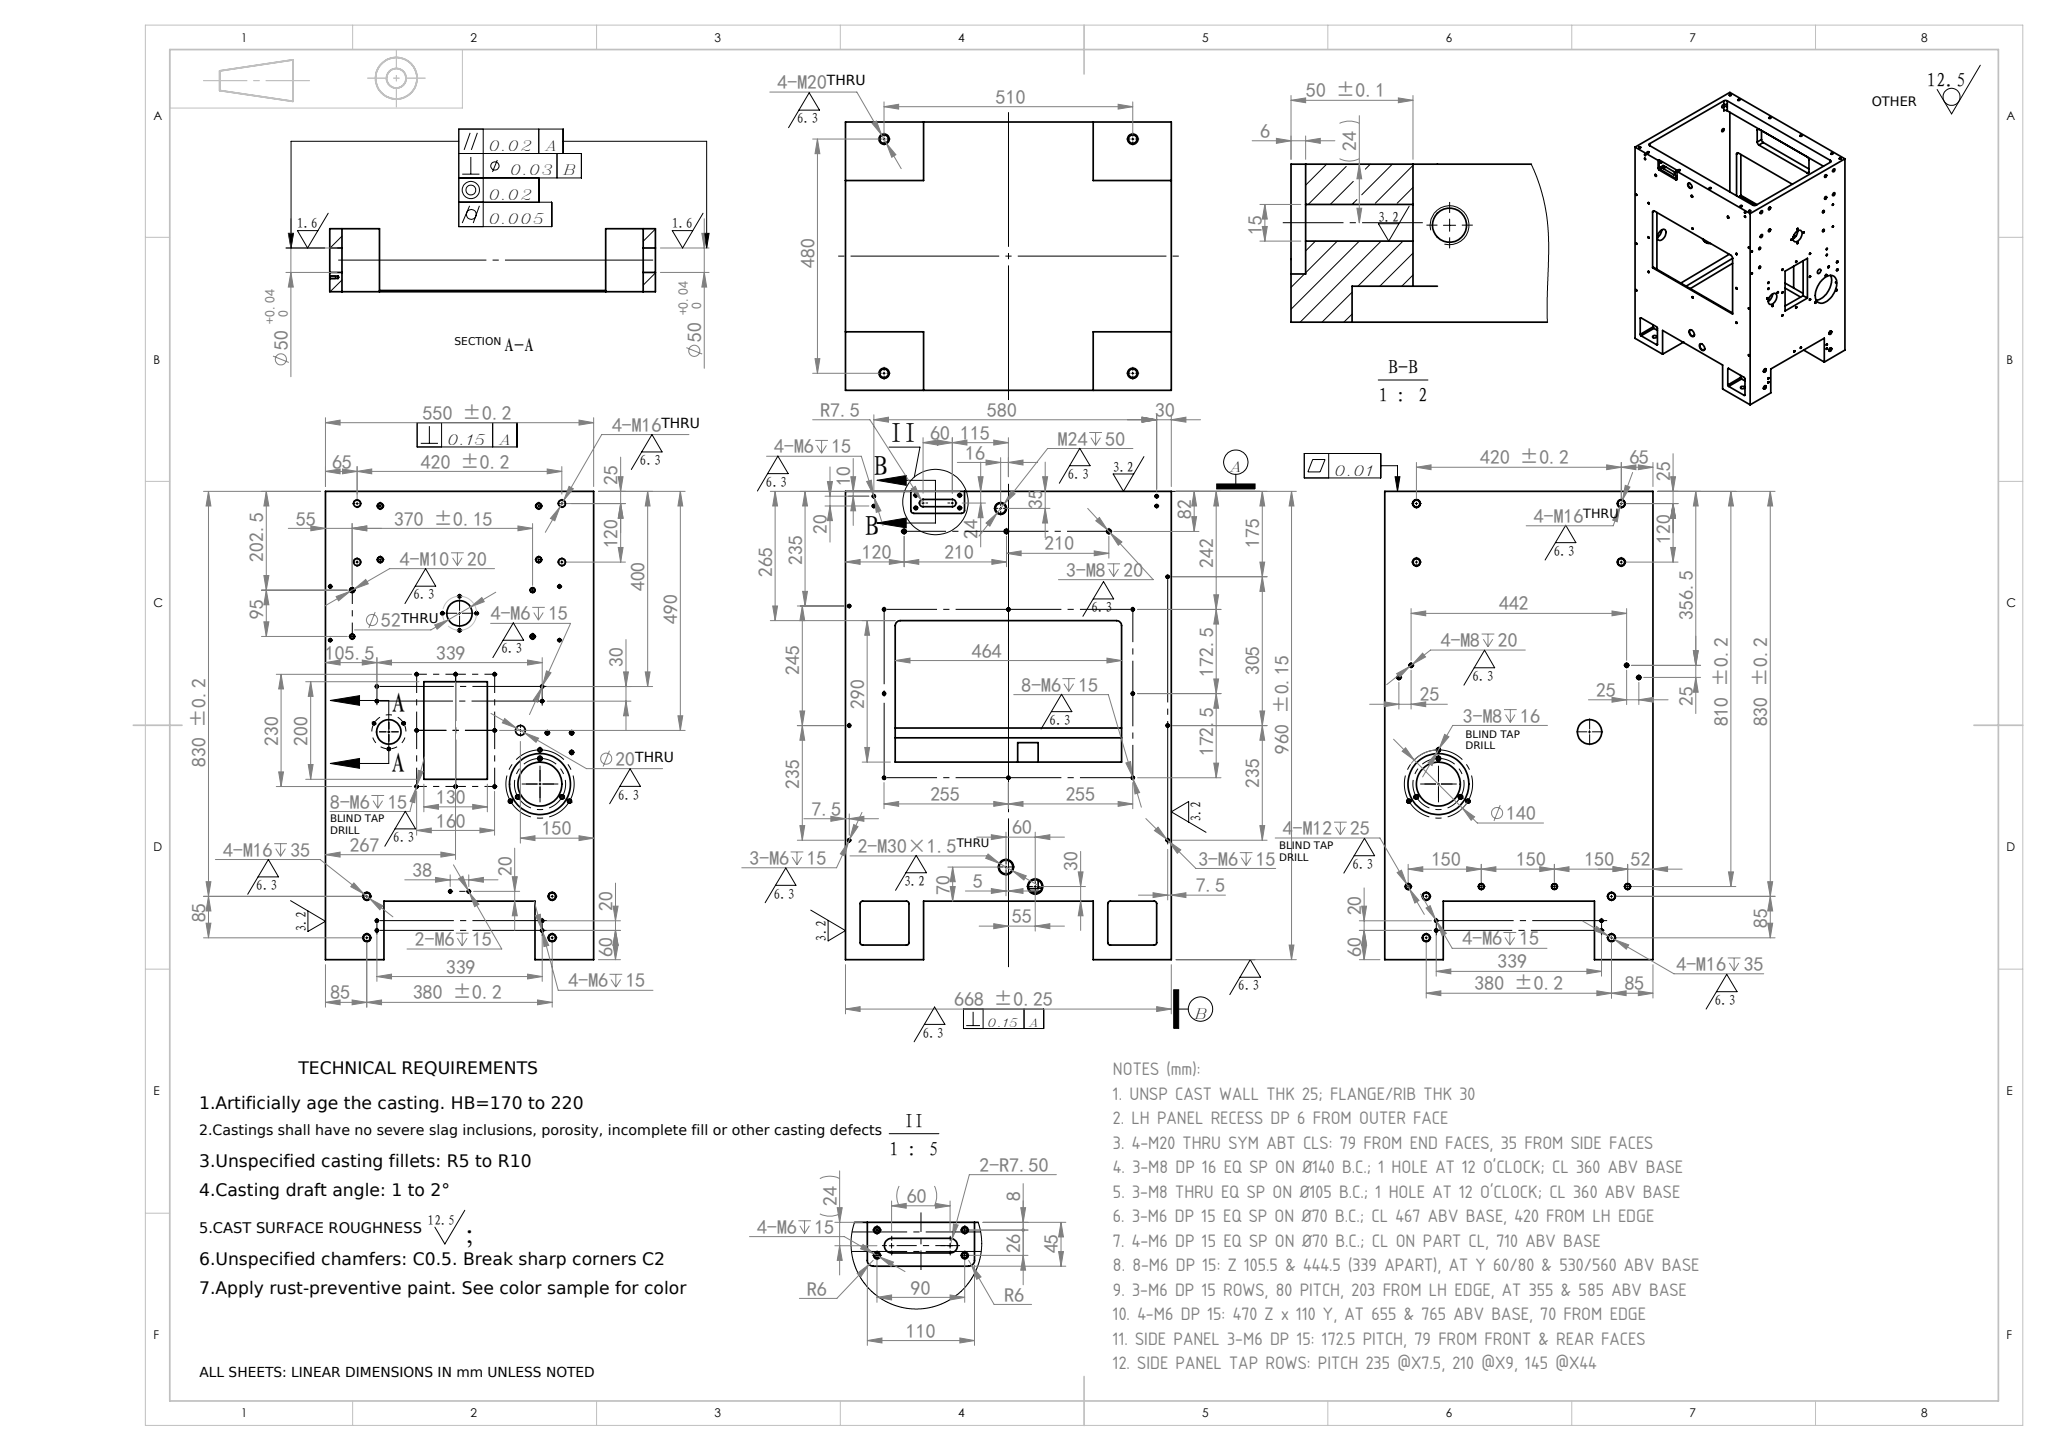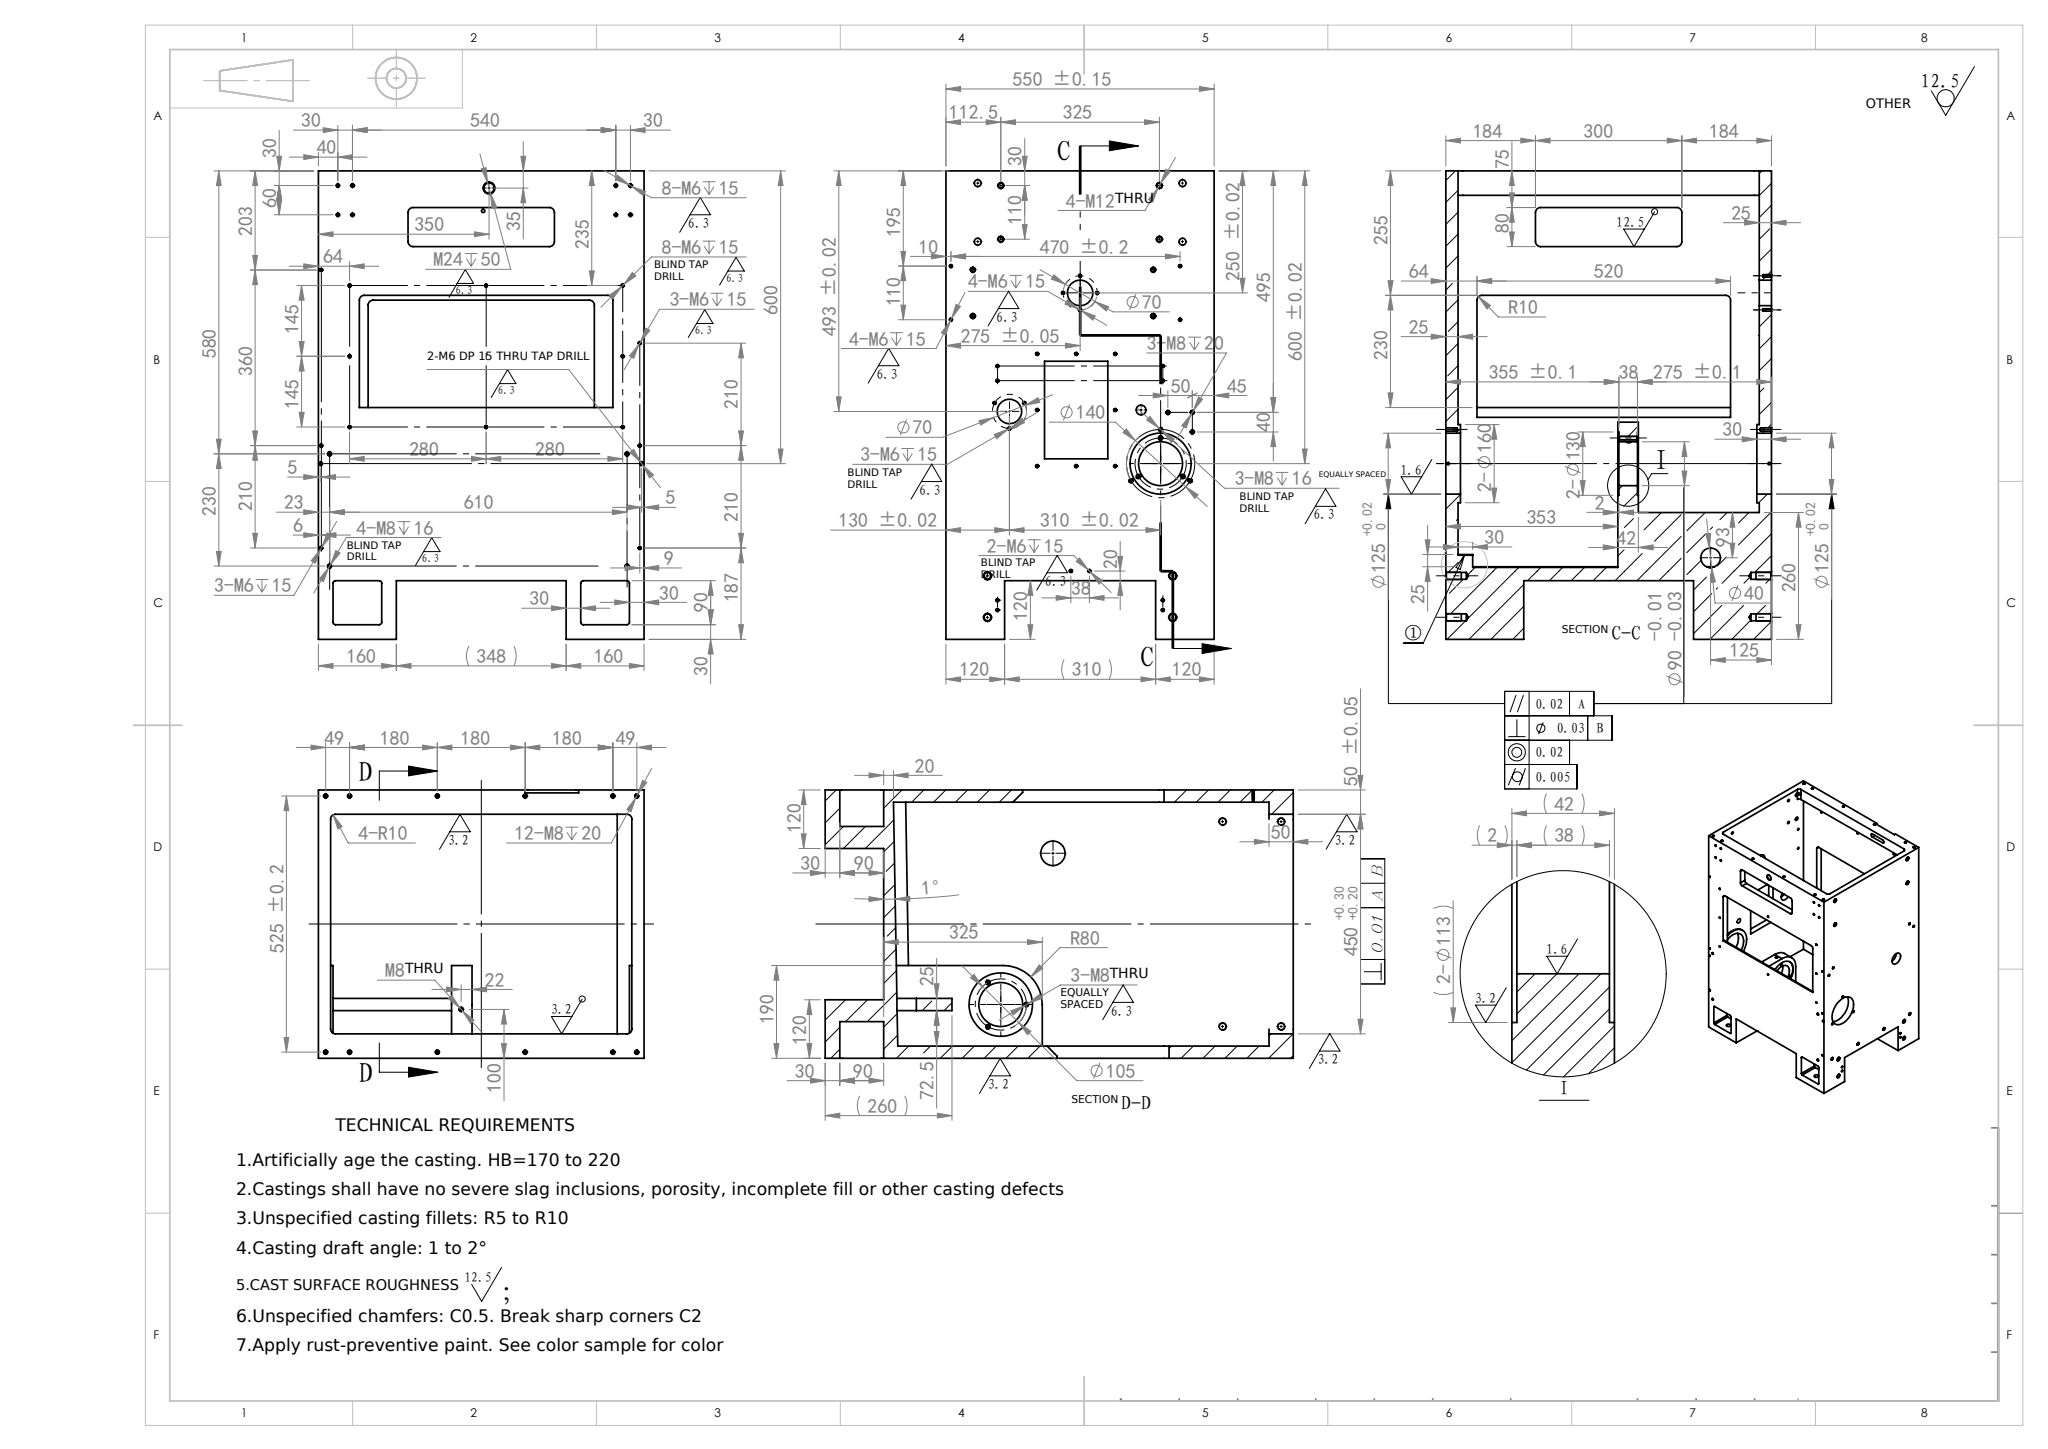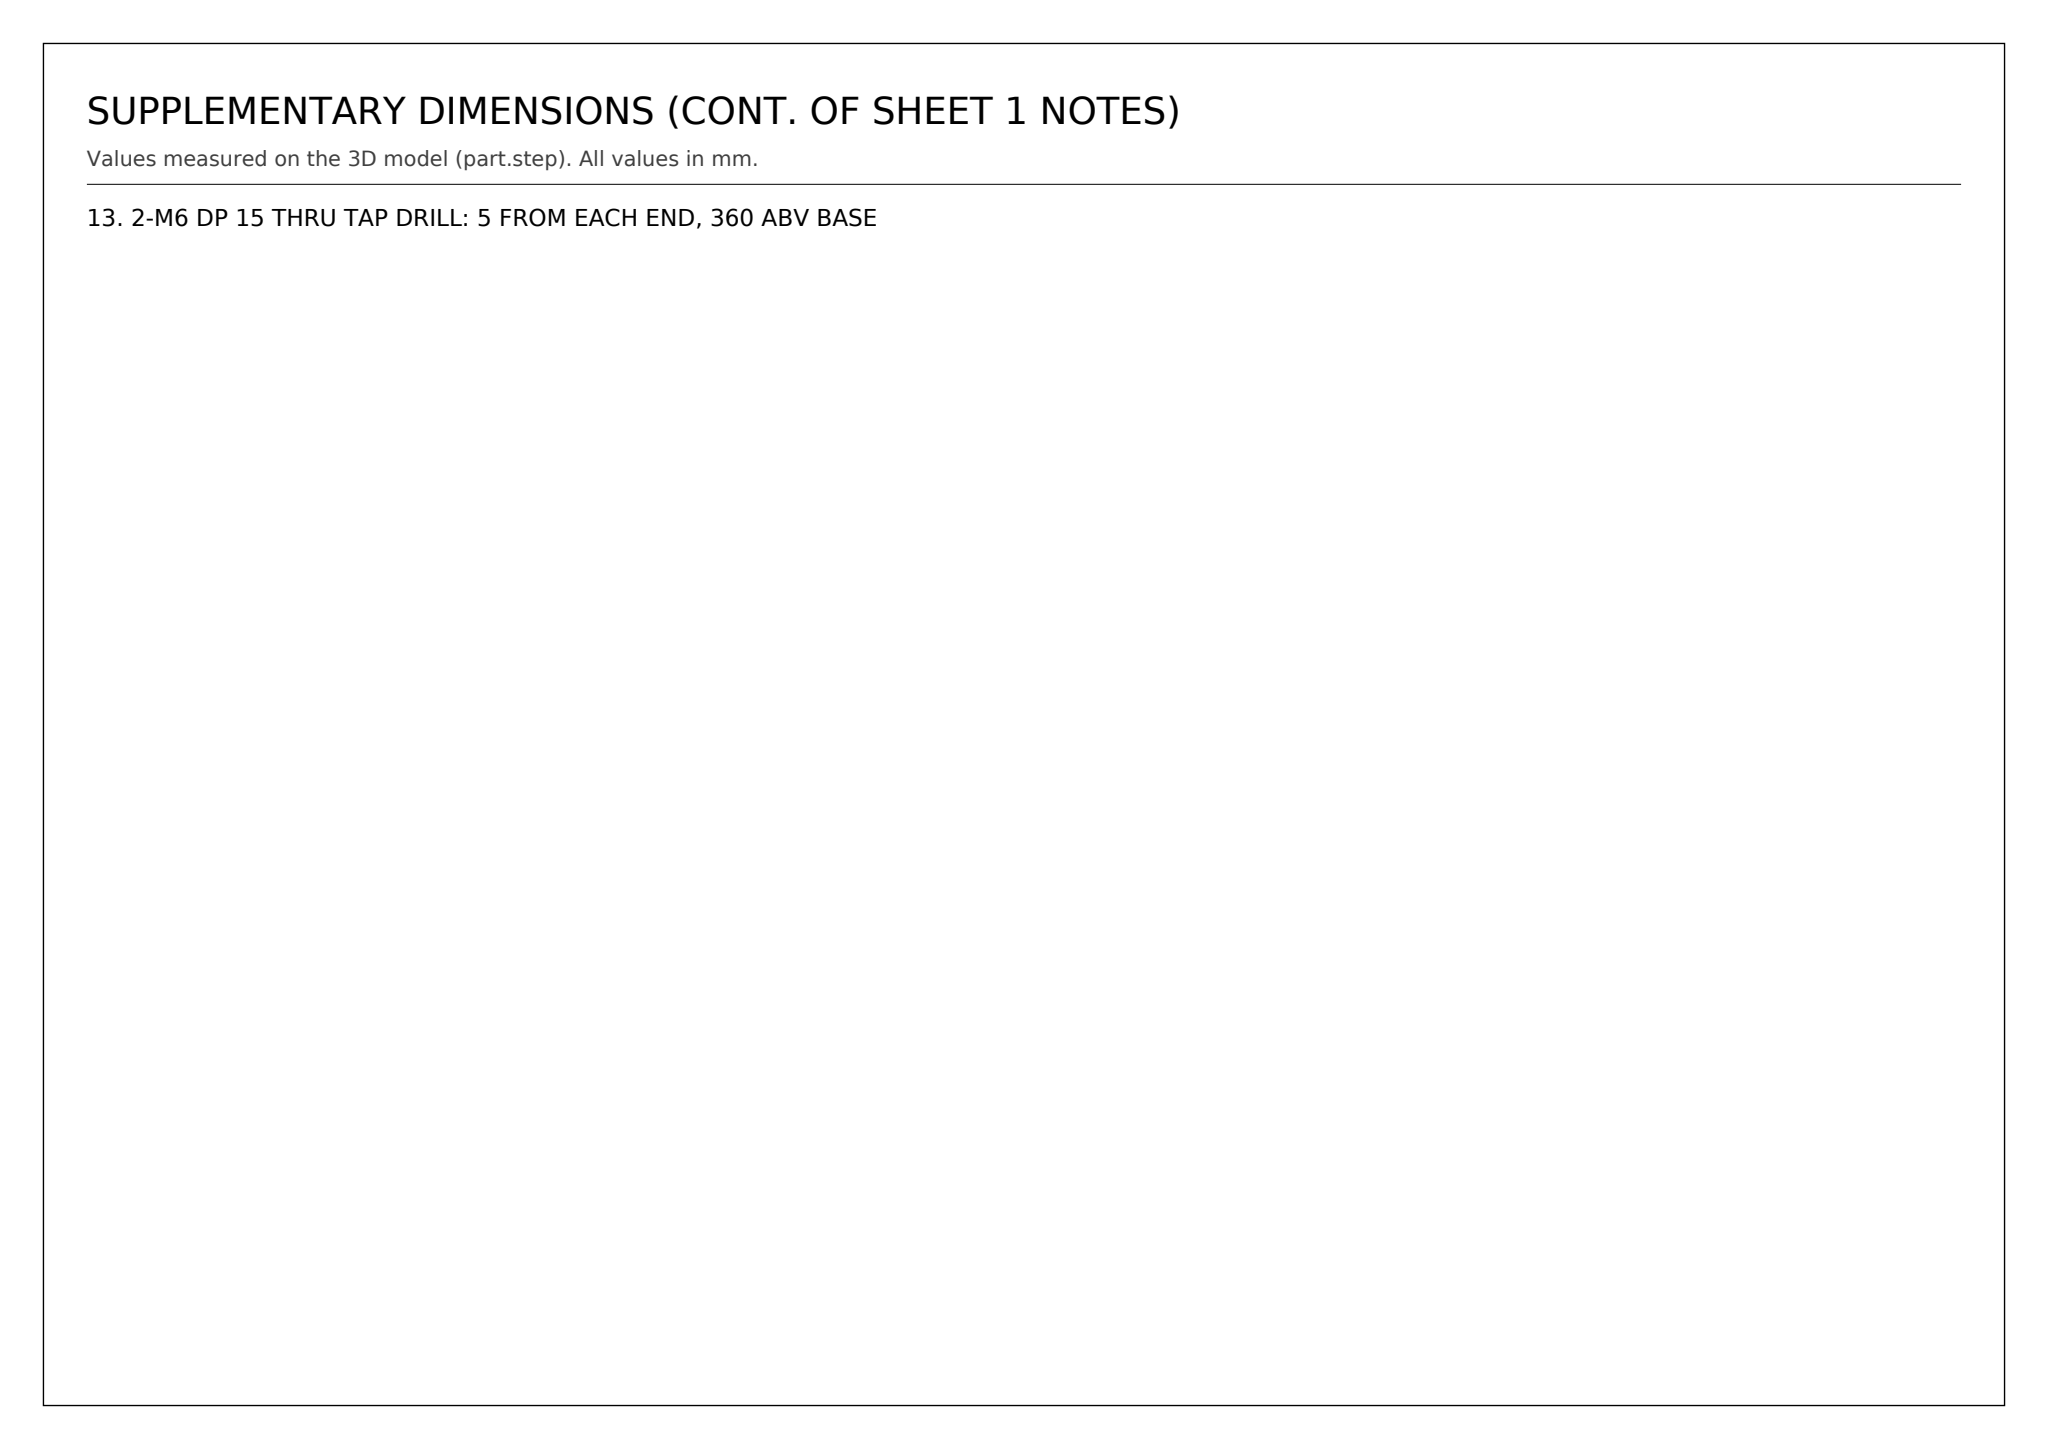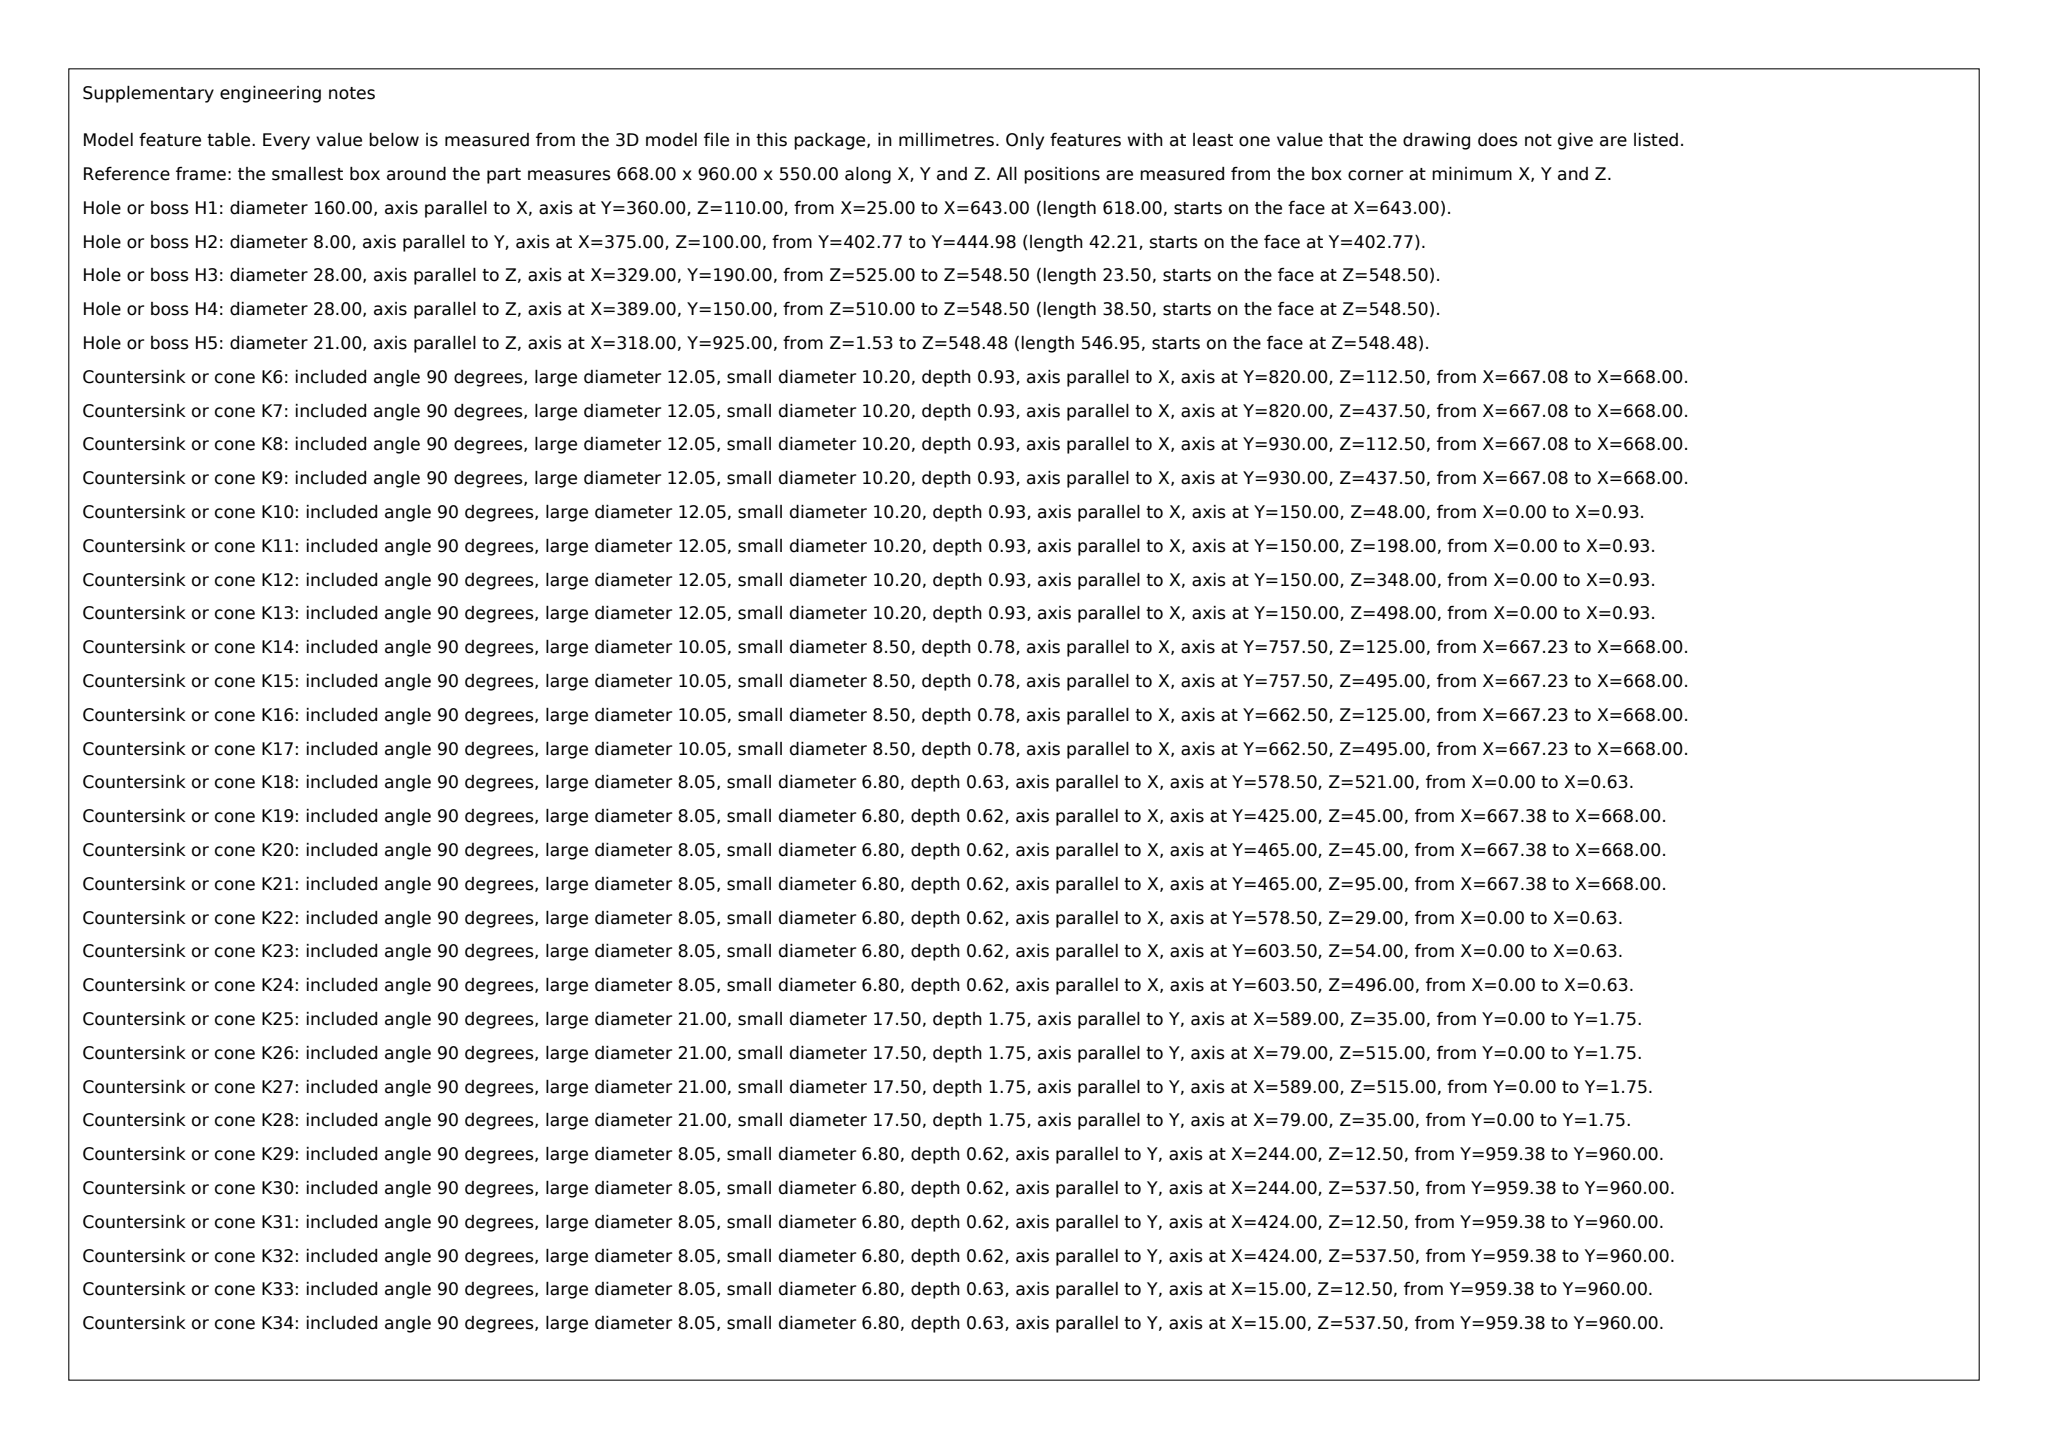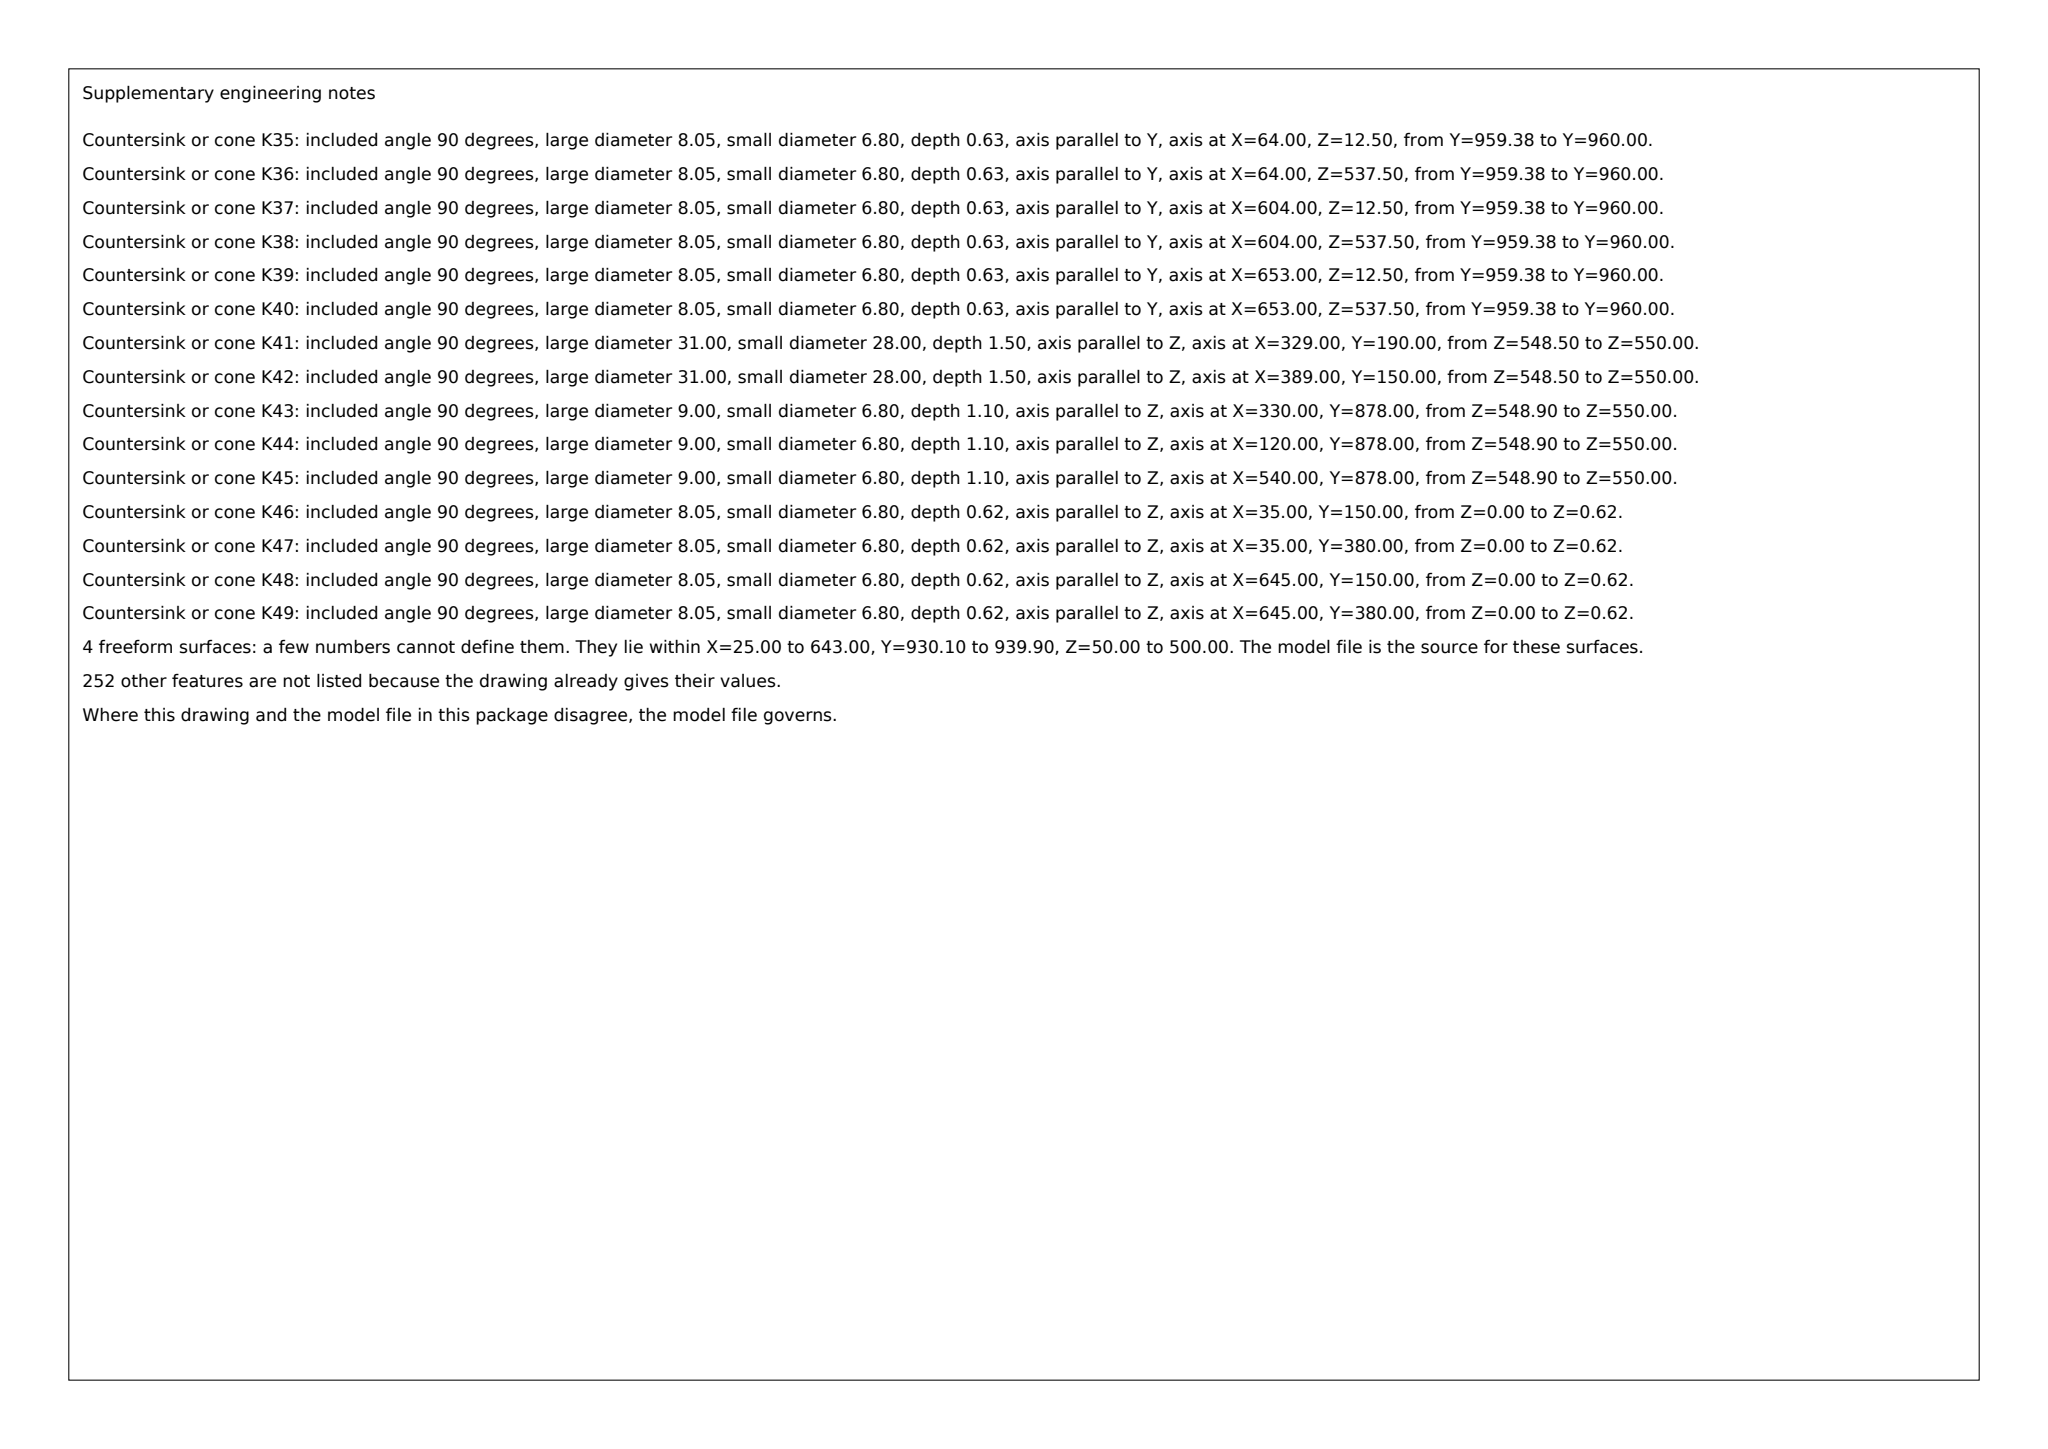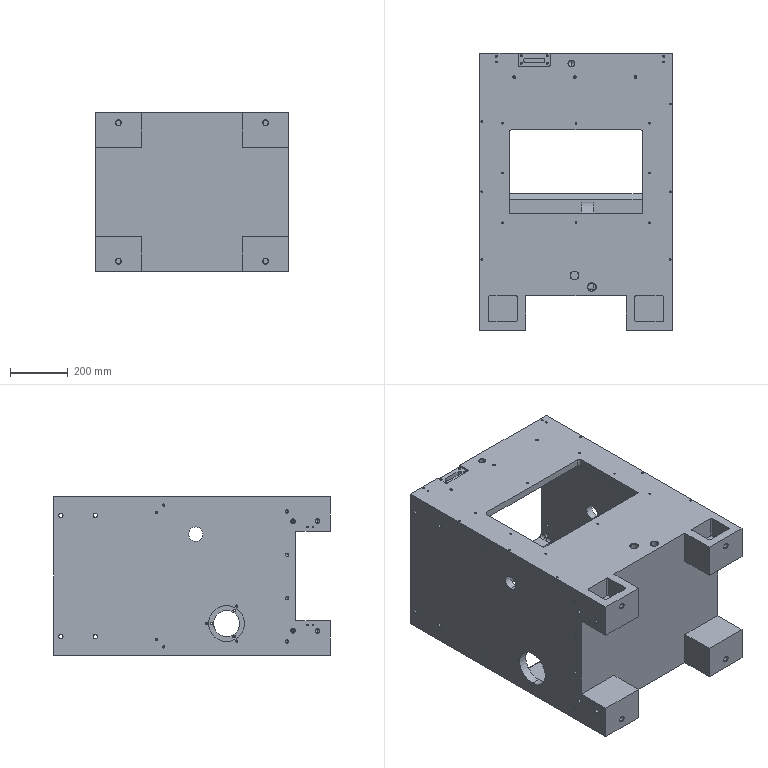Part | SolidWorks | mm | 1 solid | 997 faces | box 668 x 960 x 550 mm | volume 58582105 mm3 | cone 542 | cylinder 364 | plane 87 | spline 4 | commonest cylinder face diameters 5 x158 6.8 x70 14 x32 20 x18 10.2 x16 10 x16 8.5 x8 17.5 x8
Drawing notes:
UNSP CAST WALL THK 25; FLANGE/RIB THK 30 | from the solid: x planes 0/25 & 643/668 (25); x planes 30 & 638 (30); z planes 0/25 and 525/550
LH PANEL RECESS DP 6 FROM OUTER FACE | from the solid: z planes 550 (outer face) and 544
4-M20 THRU SYM ABT CLS: 79 FROM END FACES, 35 FROM SIDE FACES | from the solid: bbox 668 x 550 with 510 x 480 pattern on CLs: (668-510)/2=79, (550-480)/2=35
3-M8 DP 16 EQ SP ON Ø140 B.C.; 1 HOLE AT 12 O'CLOCK; CL 360 ABV BASE | from the solid: Ø6.8 x-axis tap drills (Y325,Z49.38),(Y325,Z170.62) chord 121.24 -> R70 abt Y360/Z110
3-M8 THRU EQ SP ON Ø105 B.C.; 1 HOLE AT 12 O'CLOCK; CL 360 ABV BASE | from the solid: Ø6.8 thru holes L35.8 at (Y333.75,Z64.53),(Y333.75,Z155.47),(Y412.5,Z110), R52.5
3-M6 DP 15 EQ SP ON Ø70 B.C.; CL 467 ABV BASE, 420 FROM LH EDGE | from the solid: Ø5 x-axis taps (432,420),(484.5,389.69),(484.5,450.31) = R35 abt (467,420)
4-M6 DP 15 EQ SP ON Ø70 B.C.; CL ON PART CL, 710 ABV BASE | from the solid: Ø5 x-axis taps (675,275),(710,240),(710,310),(745,275) = R35 abt (710,275)
8-M6 DP 15: Z 105.5 & 444.5 (339 APART), AT Y 60/80 & 530/560 ABV BASE | from the solid: Ø5 x-axis taps y60/80 and y530/560 at z105.5 & z444.5, len 19.48
3-M6 DP 15 ROWS, 80 PITCH, 203 FROM LH EDGE, AT 355 & 585 ABV BASE | from the solid: Ø5 x-axis taps (y355,z203/283/363) and (y585,z203/283/363), len 16.48
4-M6 DP 15: 470 Z x 110 Y, AT 655 & 765 ABV BASE, 70 FROM EDGE | from the solid: Ø5 x-axis taps (655,70),(655,540),(765,70),(765,540), len 16.48
SIDE PANEL 3-M6 DP 15: 172.5 PITCH, 79 FROM FRONT & REAR FACES | from the solid: Ø5 z-axis taps x79 & x589, y373/545.5/718, len 16.48
SIDE PANEL TAP ROWS: PITCH 235 @X7.5, 210 @X9, 145 @X44 | from the solid: Ø5 z-taps x7.5 y245/480/725; x9 y187/397/607; x44 y435/580/725
2-M6 DP 15 THRU TAP DRILL: 5 FROM EACH END, 360 ABV BASE | from the solid: Ø5 z-axis holes (X5,Y360) and (X663,Y360), L46.55 thru side panel; X bbox 668